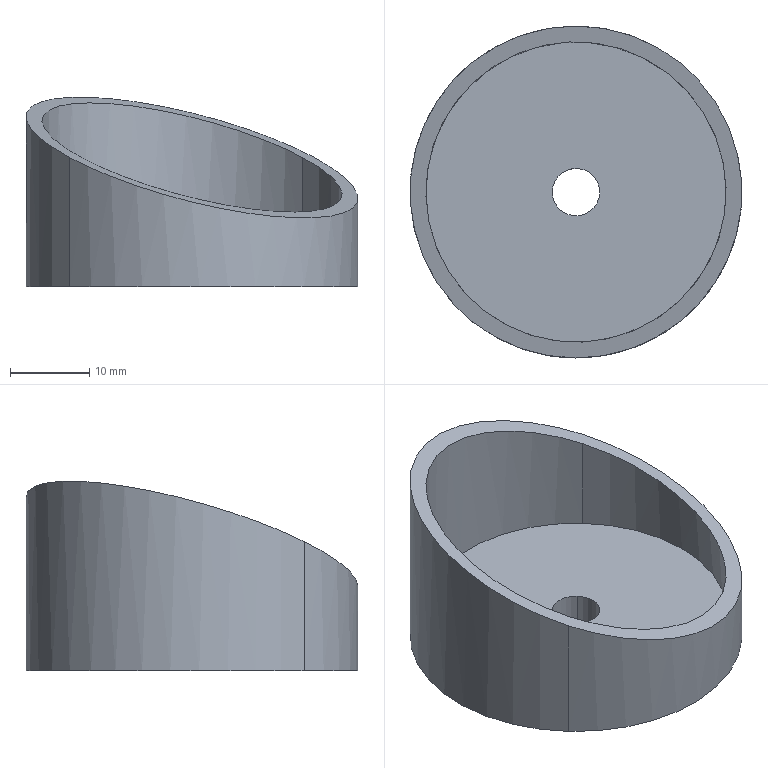Component | SolidWorks | Cam2-1 | 1 solid | 9 faces | box 42 x 42 x 24 mm | volume 8534 mm3 | cylinder 6 | plane 3 | commonest cylinder face diameters 6 x2 38 x2 42 x2
build123d program:
from build123d import *

# Parameters (mm, degrees)
SKETCH1_R           = 21
SKETCH1_R_2         = 19
BOSS_EXTRUDE1_DEPTH = 20
BOSS_EXTRUDE2_START = 4
SKETCH2_R           = 21
SKETCH2_R_2         = 3
BOSS_EXTRUDE2_DEPTH = 4
CUT_EXTRUDE1_DEPTH  = 45.5


with BuildPart() as part:
    # Sketch1 → Boss-Extrude1 (new body)
    with BuildSketch(Plane(origin=(0, 0, 0), x_dir=(1, 0, 0), z_dir=(0, 1, 0))):
        with Locations(Location((0, 0, 0), (0, 0, 270))):
            Circle(SKETCH1_R)
        with Locations(Location((0, 0, 0), (0, 0, 270))):
            Circle(SKETCH1_R_2, mode=Mode.SUBTRACT)
    extrude(amount=BOSS_EXTRUDE1_DEPTH)

    # Sketch2 → Boss-Extrude2 (add)
    with BuildSketch(Plane.XZ.offset(BOSS_EXTRUDE2_START)):
        with Locations(Location((0, 0, 0), (0, 0, 270))):
            Circle(SKETCH2_R)
        with Locations(Location((0, 0, 0), (0, 0, 270))):
            Circle(SKETCH2_R_2, mode=Mode.SUBTRACT)
    extrude(amount=-BOSS_EXTRUDE2_DEPTH)

    # Sketch3 → Cut-Extrude1 (cut, symmetric)
    with BuildSketch(Plane.XY):
        Polygon((-21, 4.713), (21, 20), (-22.824, 41.392), align=None)
    extrude(amount=CUT_EXTRUDE1_DEPTH, both=True, mode=Mode.SUBTRACT)


solid = part.part

# Placed as in the assembly
solid = solid.moved(Location((-15.928, -1.7, 15.655), (-90, 47.49, 179.998)))
STEP:
#1=COLOUR_RGB('',0.7922,0.8196,0.9333);
#2=FILL_AREA_STYLE_COLOUR('',#1);
#3=FILL_AREA_STYLE('',(#2));
#4=SURFACE_STYLE_FILL_AREA(#3);
#5=SURFACE_SIDE_STYLE('',(#4));
#6=SURFACE_STYLE_USAGE(.BOTH.,#5);
#7=PRESENTATION_STYLE_ASSIGNMENT((#6));
#8=CARTESIAN_POINT('',(-0.54,0.01287,0.4589));
#9=VERTEX_POINT('',#8);
#10=CARTESIAN_POINT('',(-0.7142,-0.1467,0.4589));
#11=VERTEX_POINT('',#10);
#12=CARTESIAN_POINT('',(-0.6271,-0.06694,0.4589));
#13=DIRECTION('',(0.,0.,-1.));
#14=DIRECTION('',(-0.7372,-0.6757,0.));
#15=AXIS2_PLACEMENT_3D('',#12,#13,#14);
#16=CIRCLE('',#15,0.1181);
#17=EDGE_CURVE('',#9,#11,#16,.T.);
#18=ORIENTED_EDGE('',*,*,#17,.T.);
#19=CARTESIAN_POINT('',(-0.7142,-0.1467,0.6163));
#20=VERTEX_POINT('',#19);
#21=CARTESIAN_POINT('',(-0.7142,-0.1467,0.4589));
#22=DIRECTION('',(0.,0.,1.));
#23=VECTOR('',#22,39.37);
#24=LINE('',#21,#23);
#25=EDGE_CURVE('',#11,#20,#24,.T.);
#26=ORIENTED_EDGE('',*,*,#25,.T.);
#27=CARTESIAN_POINT('',(-0.54,0.01287,0.6163));
#28=VERTEX_POINT('',#27);
#29=CARTESIAN_POINT('',(-0.6271,-0.06694,0.6163));
#30=DIRECTION('',(0.,0.,-1.));
#31=DIRECTION('',(-0.7372,-0.6757,0.));
#32=AXIS2_PLACEMENT_3D('',#29,#30,#31);
#33=CIRCLE('',#32,0.1181);
#34=EDGE_CURVE('',#28,#20,#33,.T.);
#35=ORIENTED_EDGE('',*,*,#34,.F.);
#36=CARTESIAN_POINT('',(-0.54,0.01287,0.4589));
#37=DIRECTION('',(0.,0.,1.));
#38=VECTOR('',#37,39.37);
#39=LINE('',#36,#38);
#40=EDGE_CURVE('',#9,#28,#39,.T.);
#41=ORIENTED_EDGE('',*,*,#40,.F.);
#42=EDGE_LOOP('',(#18,#26,#35,#41));
#43=FACE_OUTER_BOUND('',#42,.T.);
#44=CARTESIAN_POINT('',(-0.6271,-0.06694,0.4589));
#45=DIRECTION('',(0.,0.,1.));
#46=DIRECTION('',(0.7372,0.6757,0.));
#47=AXIS2_PLACEMENT_3D('',#44,#45,#46);
#48=CYLINDRICAL_SURFACE('',#47,0.1181);
#49=ADVANCED_FACE('',(#43),#48,.F.);
#50=CARTESIAN_POINT('',(-0.07567,0.4385,1.103));
#51=VERTEX_POINT('',#50);
#52=CARTESIAN_POINT('',(-1.179,-0.5724,1.103));
#53=VERTEX_POINT('',#52);
#54=CARTESIAN_POINT('',(-0.07567,0.4385,1.103));
#55=CARTESIAN_POINT('',(0.9353,-0.6643,0.5583));
#56=CARTESIAN_POINT('',(-0.1676,-1.675,0.5583));
#57=CARTESIAN_POINT('',(-1.179,-0.5724,1.103));
#58=(BOUNDED_CURVE()B_SPLINE_CURVE(3,(#54,#55,#56,#57),.UNSPECIFIED.,.F.,.F.)B_SPLINE_CURVE_WITH_KNOTS((4,4),(4.712,7.854),.UNSPECIFIED.)CURVE()GEOMETRIC_REPRESENTATION_ITEM()RATIONAL_B_SPLINE_CURVE((1.,0.3333,0.3333,1.))REPRESENTATION_ITEM(''));
#59=EDGE_CURVE('',#51,#53,#58,.T.);
#60=ORIENTED_EDGE('',*,*,#59,.F.);
#61=CARTESIAN_POINT('',(-0.07567,0.4385,0.6163));
#62=VERTEX_POINT('',#61);
#63=CARTESIAN_POINT('',(-0.07567,0.4385,1.404));
#64=DIRECTION('',(0.,0.,-1.));
#65=VECTOR('',#64,39.37);
#66=LINE('',#63,#65);
#67=EDGE_CURVE('',#51,#62,#66,.T.);
#68=ORIENTED_EDGE('',*,*,#67,.T.);
#69=CARTESIAN_POINT('',(-1.179,-0.5724,0.6163));
#70=VERTEX_POINT('',#69);
#71=CARTESIAN_POINT('',(-0.6271,-0.06694,0.6163));
#72=DIRECTION('',(0.,0.,1.));
#73=DIRECTION('',(0.7372,0.6757,0.));
#74=AXIS2_PLACEMENT_3D('',#71,#72,#73);
#75=CIRCLE('',#74,0.748);
#76=EDGE_CURVE('',#70,#62,#75,.T.);
#77=ORIENTED_EDGE('',*,*,#76,.F.);
#78=CARTESIAN_POINT('',(-1.179,-0.5724,1.404));
#79=DIRECTION('',(0.,0.,-1.));
#80=VECTOR('',#79,39.37);
#81=LINE('',#78,#80);
#82=EDGE_CURVE('',#53,#70,#81,.T.);
#83=ORIENTED_EDGE('',*,*,#82,.F.);
#84=EDGE_LOOP('',(#60,#68,#77,#83));
#85=FACE_OUTER_BOUND('',#84,.T.);
#86=CARTESIAN_POINT('',(-0.6271,-0.06694,1.404));
#87=DIRECTION('',(0.,0.,-1.));
#88=DIRECTION('',(-0.7372,-0.6757,0.));
#89=AXIS2_PLACEMENT_3D('',#86,#87,#88);
#90=CYLINDRICAL_SURFACE('',#89,0.748);
#91=ADVANCED_FACE('',(#85),#90,.F.);
#92=CARTESIAN_POINT('',(-1.237,-0.6256,1.103));
#93=VERTEX_POINT('',#92);
#94=CARTESIAN_POINT('',(-0.01763,0.4917,1.103));
#95=VERTEX_POINT('',#94);
#96=CARTESIAN_POINT('',(-1.237,-0.6256,1.103));
#97=CARTESIAN_POINT('',(-2.354,0.5933,1.705));
#98=CARTESIAN_POINT('',(-1.135,1.711,1.705));
#99=CARTESIAN_POINT('',(-0.01763,0.4917,1.103));
#100=(BOUNDED_CURVE()B_SPLINE_CURVE(3,(#96,#97,#98,#99),.UNSPECIFIED.,.F.,.T.)B_SPLINE_CURVE_WITH_KNOTS((4,4),(1.571,4.712),.UNSPECIFIED.)CURVE()GEOMETRIC_REPRESENTATION_ITEM()RATIONAL_B_SPLINE_CURVE((1.,0.3333,0.3333,1.))REPRESENTATION_ITEM(''));
#101=EDGE_CURVE('',#93,#95,#100,.T.);
#102=ORIENTED_EDGE('',*,*,#101,.T.);
#103=CARTESIAN_POINT('',(-0.01763,0.4917,0.4589));
#104=VERTEX_POINT('',#103);
#105=CARTESIAN_POINT('',(-0.01763,0.4917,1.404));
#106=DIRECTION('',(0.,0.,-1.));
#107=VECTOR('',#106,39.37);
#108=LINE('',#105,#107);
#109=EDGE_CURVE('',#95,#104,#108,.T.);
#110=ORIENTED_EDGE('',*,*,#109,.T.);
#111=CARTESIAN_POINT('',(-1.237,-0.6256,0.4589));
#112=VERTEX_POINT('',#111);
#113=CARTESIAN_POINT('',(-0.6271,-0.06694,0.4589));
#114=DIRECTION('',(0.,0.,-1.));
#115=DIRECTION('',(-0.7372,-0.6757,0.));
#116=AXIS2_PLACEMENT_3D('',#113,#114,#115);
#117=CIRCLE('',#116,0.8268);
#118=EDGE_CURVE('',#112,#104,#117,.T.);
#119=ORIENTED_EDGE('',*,*,#118,.F.);
#120=CARTESIAN_POINT('',(-1.237,-0.6256,1.404));
#121=DIRECTION('',(0.,0.,-1.));
#122=VECTOR('',#121,39.37);
#123=LINE('',#120,#122);
#124=EDGE_CURVE('',#93,#112,#123,.T.);
#125=ORIENTED_EDGE('',*,*,#124,.F.);
#126=EDGE_LOOP('',(#102,#110,#119,#125));
#127=FACE_OUTER_BOUND('',#126,.T.);
#128=CARTESIAN_POINT('',(-0.6271,-0.06694,1.404));
#129=DIRECTION('',(0.,0.,-1.));
#130=DIRECTION('',(-0.7372,-0.6757,0.));
#131=AXIS2_PLACEMENT_3D('',#128,#129,#130);
#132=CYLINDRICAL_SURFACE('',#131,0.8268);
#133=ADVANCED_FACE('',(#127),#132,.T.);
#134=ORIENTED_EDGE('',*,*,#109,.F.);
#135=CARTESIAN_POINT('',(-0.01763,0.4917,1.103));
#136=CARTESIAN_POINT('',(1.1,-0.7272,0.501));
#137=CARTESIAN_POINT('',(-0.1192,-1.845,0.501));
#138=CARTESIAN_POINT('',(-1.237,-0.6256,1.103));
#139=(BOUNDED_CURVE()B_SPLINE_CURVE(3,(#135,#136,#137,#138),.UNSPECIFIED.,.F.,.F.)B_SPLINE_CURVE_WITH_KNOTS((4,4),(4.712,7.854),.UNSPECIFIED.)CURVE()GEOMETRIC_REPRESENTATION_ITEM()RATIONAL_B_SPLINE_CURVE((1.,0.3333,0.3333,1.))REPRESENTATION_ITEM(''));
#140=EDGE_CURVE('',#95,#93,#139,.T.);
#141=ORIENTED_EDGE('',*,*,#140,.T.);
#142=ORIENTED_EDGE('',*,*,#124,.T.);
#143=CARTESIAN_POINT('',(-0.6271,-0.06694,0.4589));
#144=DIRECTION('',(0.,0.,-1.));
#145=DIRECTION('',(-0.7372,-0.6757,0.));
#146=AXIS2_PLACEMENT_3D('',#143,#144,#145);
#147=CIRCLE('',#146,0.8268);
#148=EDGE_CURVE('',#104,#112,#147,.T.);
#149=ORIENTED_EDGE('',*,*,#148,.F.);
#150=EDGE_LOOP('',(#134,#141,#142,#149));
#151=FACE_OUTER_BOUND('',#150,.T.);
#152=CARTESIAN_POINT('',(-0.6271,-0.06694,1.404));
#153=DIRECTION('',(0.,0.,-1.));
#154=DIRECTION('',(-0.7372,-0.6757,0.));
#155=AXIS2_PLACEMENT_3D('',#152,#153,#154);
#156=CYLINDRICAL_SURFACE('',#155,0.8268);
#157=ADVANCED_FACE('',(#151),#156,.T.);
#158=ORIENTED_EDGE('',*,*,#67,.F.);
#159=CARTESIAN_POINT('',(-1.179,-0.5724,1.103));
#160=CARTESIAN_POINT('',(-2.189,0.5304,1.647));
#161=CARTESIAN_POINT('',(-1.087,1.541,1.647));
#162=CARTESIAN_POINT('',(-0.07567,0.4385,1.103));
#163=(BOUNDED_CURVE()B_SPLINE_CURVE(3,(#159,#160,#161,#162),.UNSPECIFIED.,.F.,.F.)B_SPLINE_CURVE_WITH_KNOTS((4,4),(1.571,4.712),.UNSPECIFIED.)CURVE()GEOMETRIC_REPRESENTATION_ITEM()RATIONAL_B_SPLINE_CURVE((1.,0.3333,0.3333,1.))REPRESENTATION_ITEM(''));
#164=EDGE_CURVE('',#53,#51,#163,.T.);
#165=ORIENTED_EDGE('',*,*,#164,.F.);
#166=ORIENTED_EDGE('',*,*,#82,.T.);
#167=CARTESIAN_POINT('',(-0.6271,-0.06694,0.6163));
#168=DIRECTION('',(0.,0.,1.));
#169=DIRECTION('',(0.7372,0.6757,0.));
#170=AXIS2_PLACEMENT_3D('',#167,#168,#169);
#171=CIRCLE('',#170,0.748);
#172=EDGE_CURVE('',#62,#70,#171,.T.);
#173=ORIENTED_EDGE('',*,*,#172,.F.);
#174=EDGE_LOOP('',(#158,#165,#166,#173));
#175=FACE_OUTER_BOUND('',#174,.T.);
#176=CARTESIAN_POINT('',(-0.6271,-0.06694,1.404));
#177=DIRECTION('',(0.,0.,-1.));
#178=DIRECTION('',(-0.7372,-0.6757,0.));
#179=AXIS2_PLACEMENT_3D('',#176,#177,#178);
#180=CYLINDRICAL_SURFACE('',#179,0.748);
#181=ADVANCED_FACE('',(#175),#180,.F.);
#182=ORIENTED_EDGE('',*,*,#118,.T.);
#183=ORIENTED_EDGE('',*,*,#148,.T.);
#184=EDGE_LOOP('',(#182,#183));
#185=FACE_OUTER_BOUND('',#184,.T.);
#186=ORIENTED_EDGE('',*,*,#17,.F.);
#187=CARTESIAN_POINT('',(-0.6271,-0.06694,0.4589));
#188=DIRECTION('',(0.,0.,-1.));
#189=DIRECTION('',(-0.7372,-0.6757,0.));
#190=AXIS2_PLACEMENT_3D('',#187,#188,#189);
#191=CIRCLE('',#190,0.1181);
#192=EDGE_CURVE('',#11,#9,#191,.T.);
#193=ORIENTED_EDGE('',*,*,#192,.F.);
#194=EDGE_LOOP('',(#186,#193));
#195=FACE_BOUND('',#194,.T.);
#196=CARTESIAN_POINT('',(-0.6271,-0.06694,0.4589));
#197=DIRECTION('',(0.,0.,-1.));
#198=DIRECTION('',(-0.7372,-0.6757,0.));
#199=AXIS2_PLACEMENT_3D('',#196,#197,#198);
#200=PLANE('',#199);
#201=ADVANCED_FACE('',(#185,#195),#200,.T.);
#202=ORIENTED_EDGE('',*,*,#76,.T.);
#203=ORIENTED_EDGE('',*,*,#172,.T.);
#204=EDGE_LOOP('',(#202,#203));
#205=FACE_OUTER_BOUND('',#204,.T.);
#206=ORIENTED_EDGE('',*,*,#34,.T.);
#207=CARTESIAN_POINT('',(-0.6271,-0.06694,0.6163));
#208=DIRECTION('',(0.,0.,-1.));
#209=DIRECTION('',(-0.7372,-0.6757,0.));
#210=AXIS2_PLACEMENT_3D('',#207,#208,#209);
#211=CIRCLE('',#210,0.1181);
#212=EDGE_CURVE('',#20,#28,#211,.T.);
#213=ORIENTED_EDGE('',*,*,#212,.T.);
#214=EDGE_LOOP('',(#206,#213));
#215=FACE_BOUND('',#214,.T.);
#216=CARTESIAN_POINT('',(-0.6271,-0.06694,0.6163));
#217=DIRECTION('',(0.,0.,-1.));
#218=DIRECTION('',(-0.7372,-0.6757,0.));
#219=AXIS2_PLACEMENT_3D('',#216,#217,#218);
#220=PLANE('',#219);
#221=ADVANCED_FACE('',(#205,#215),#220,.F.);
#222=ORIENTED_EDGE('',*,*,#25,.F.);
#223=ORIENTED_EDGE('',*,*,#192,.T.);
#224=ORIENTED_EDGE('',*,*,#40,.T.);
#225=ORIENTED_EDGE('',*,*,#212,.F.);
#226=EDGE_LOOP('',(#222,#223,#224,#225));
#227=FACE_OUTER_BOUND('',#226,.T.);
#228=CARTESIAN_POINT('',(-0.6271,-0.06694,0.4589));
#229=DIRECTION('',(0.,0.,1.));
#230=DIRECTION('',(0.7372,0.6757,0.));
#231=AXIS2_PLACEMENT_3D('',#228,#229,#230);
#232=CYLINDRICAL_SURFACE('',#231,0.1181);
#233=ADVANCED_FACE('',(#227),#232,.F.);
#234=ORIENTED_EDGE('',*,*,#164,.T.);
#235=ORIENTED_EDGE('',*,*,#59,.T.);
#236=EDGE_LOOP('',(#234,#235));
#237=FACE_BOUND('',#236,.T.);
#238=ORIENTED_EDGE('',*,*,#101,.F.);
#239=ORIENTED_EDGE('',*,*,#140,.F.);
#240=EDGE_LOOP('',(#238,#239));
#241=FACE_OUTER_BOUND('',#240,.T.);
#242=CARTESIAN_POINT('',(-1.389,-1.887,0.8019));
#243=DIRECTION('',(-0.2311,0.2521,-0.9397));
#244=DIRECTION('',(-0.635,0.6927,0.342));
#245=AXIS2_PLACEMENT_3D('',#242,#243,#244);
#246=PLANE('',#245);
#247=ADVANCED_FACE('',(#237,#241),#246,.F.);
#248=CLOSED_SHELL('',(#49,#91,#133,#157,#181,#201,#221,#233,#247));
#249=MANIFOLD_SOLID_BREP('',#248);
#250=STYLED_ITEM('',(#7),#249);
#251=PRESENTATION_LAYER_ASSIGNMENT('','',(#250));
#252=(LENGTH_UNIT()NAMED_UNIT(*)SI_UNIT($,.METRE.));
#253=LENGTH_MEASURE_WITH_UNIT(LENGTH_MEASURE(0.0254),#252);
#254=DIMENSIONAL_EXPONENTS(1.,0.,0.,0.,0.,0.,0.);
#255=(CONVERSION_BASED_UNIT('',#253)LENGTH_UNIT()NAMED_UNIT(#254));
#256=UNCERTAINTY_MEASURE_WITH_UNIT(LENGTH_MEASURE(0.00001),#255,'','');
#257=(NAMED_UNIT(*)PLANE_ANGLE_UNIT()SI_UNIT($,.RADIAN.));
#258=(NAMED_UNIT(*)SI_UNIT($,.STERADIAN.)SOLID_ANGLE_UNIT());
#259=(GEOMETRIC_REPRESENTATION_CONTEXT(3)GLOBAL_UNCERTAINTY_ASSIGNED_CONTEXT((#256))GLOBAL_UNIT_ASSIGNED_CONTEXT((#255,#257,#258))REPRESENTATION_CONTEXT('',''));
#260=MECHANICAL_DESIGN_GEOMETRIC_PRESENTATION_REPRESENTATION('',(#250),#259);
#261=CARTESIAN_POINT('',(0.,0.,0.));
#262=DIRECTION('',(0.,0.,1.));
#263=DIRECTION('',(1.,0.,0.));
#264=AXIS2_PLACEMENT_3D('',#261,#262,#263);
#265=(LENGTH_UNIT()NAMED_UNIT(*)SI_UNIT($,.METRE.));
#266=LENGTH_MEASURE_WITH_UNIT(LENGTH_MEASURE(0.0254),#265);
#267=DIMENSIONAL_EXPONENTS(1.,0.,0.,0.,0.,0.,0.);
#268=(CONVERSION_BASED_UNIT('',#266)LENGTH_UNIT()NAMED_UNIT(#267));
#269=UNCERTAINTY_MEASURE_WITH_UNIT(LENGTH_MEASURE(0.00001),#268,'','');
#270=(NAMED_UNIT(*)PLANE_ANGLE_UNIT()SI_UNIT($,.RADIAN.));
#271=(NAMED_UNIT(*)SI_UNIT($,.STERADIAN.)SOLID_ANGLE_UNIT());
#272=(GEOMETRIC_REPRESENTATION_CONTEXT(3)GLOBAL_UNCERTAINTY_ASSIGNED_CONTEXT((#269))GLOBAL_UNIT_ASSIGNED_CONTEXT((#268,#270,#271))REPRESENTATION_CONTEXT('',''));
#273=ADVANCED_BREP_SHAPE_REPRESENTATION('',(#249,#264),#272);